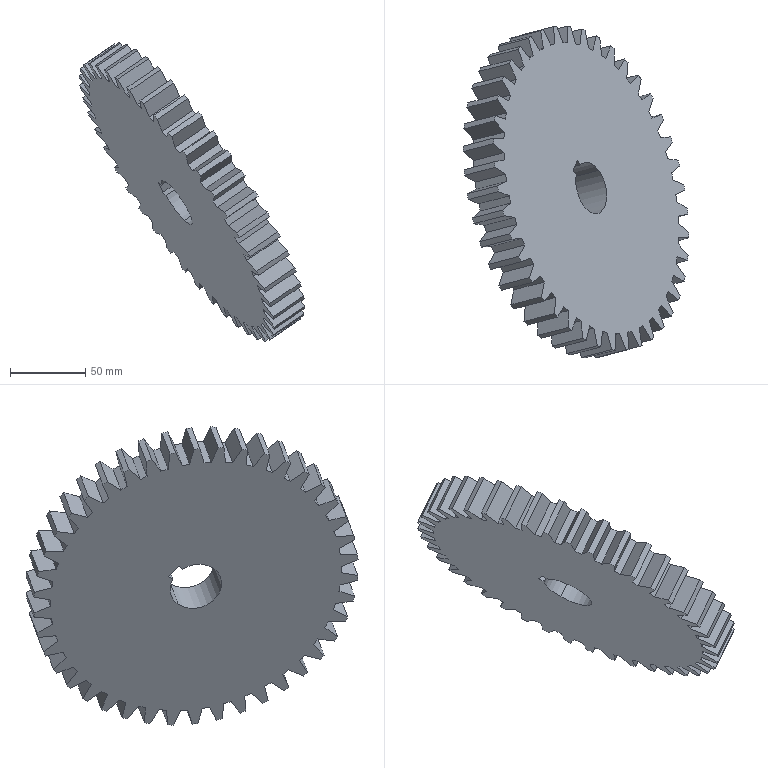Component | SolidWorks | CoarseCrusherGear-2 | 1 solid | 177 faces | box 149.59 x 220.07 x 197.55 mm | volume 819528 mm3 | plane 131 | cylinder 46 | commonest cylinder face diameters 220 x43 35 x3
build123d program:
from build123d import *

# Parameters (mm, degrees)
SKETCH1_R          = 110
SKETCH1_R_2        = 17.5
EXTRUDE1_DEPTH     = 25
CUT_EXTRUDE1_DEPTH = 25
CIRPATTERN1_COUNT  = 42
SKETCH3_W          = 10
SKETCH3_H          = 7.551
CUT_EXTRUDE2_DEPTH = 25


with BuildPart() as part:
    # Sketch1 → Extrude1 (new body)
    with BuildSketch(Plane.XY):
        Circle(SKETCH1_R)
        Circle(SKETCH1_R_2, mode=Mode.SUBTRACT)
    extrude(amount=EXTRUDE1_DEPTH)

    # Sketch2 → Cut-Extrude1 (cut)
    with BuildSketch(Plane.XY.offset(25)):
        Polygon((-6.913, 111.74), (-2.5, 98.5), (2.5, 98.5), (6.913, 111.74), align=None)
    cut_extrude1 = extrude(amount=-CUT_EXTRUDE1_DEPTH, mode=Mode.SUBTRACT)

    # CirPattern1: Cut-Extrude1 ×42 about axis
    cirpattern1_axis = Axis((0, 0, 0), (0, 0, 1))
    for i in range(1, CIRPATTERN1_COUNT):
        add(cut_extrude1.rotate(cirpattern1_axis, i * 360 / CIRPATTERN1_COUNT), mode=Mode.SUBTRACT)

    # Sketch3 → Cut-Extrude2 (cut)
    with BuildSketch(Plane.XY.offset(25)):
        with Locations((0, 17.025)):
            Rectangle(SKETCH3_W, SKETCH3_H)
    extrude(amount=-CUT_EXTRUDE2_DEPTH, mode=Mode.SUBTRACT)


solid = part.part

# Placed as in the assembly
solid = solid.moved(Location((-468.04, -178.347, -388.781), (159.138, -53.982, 119.679)))